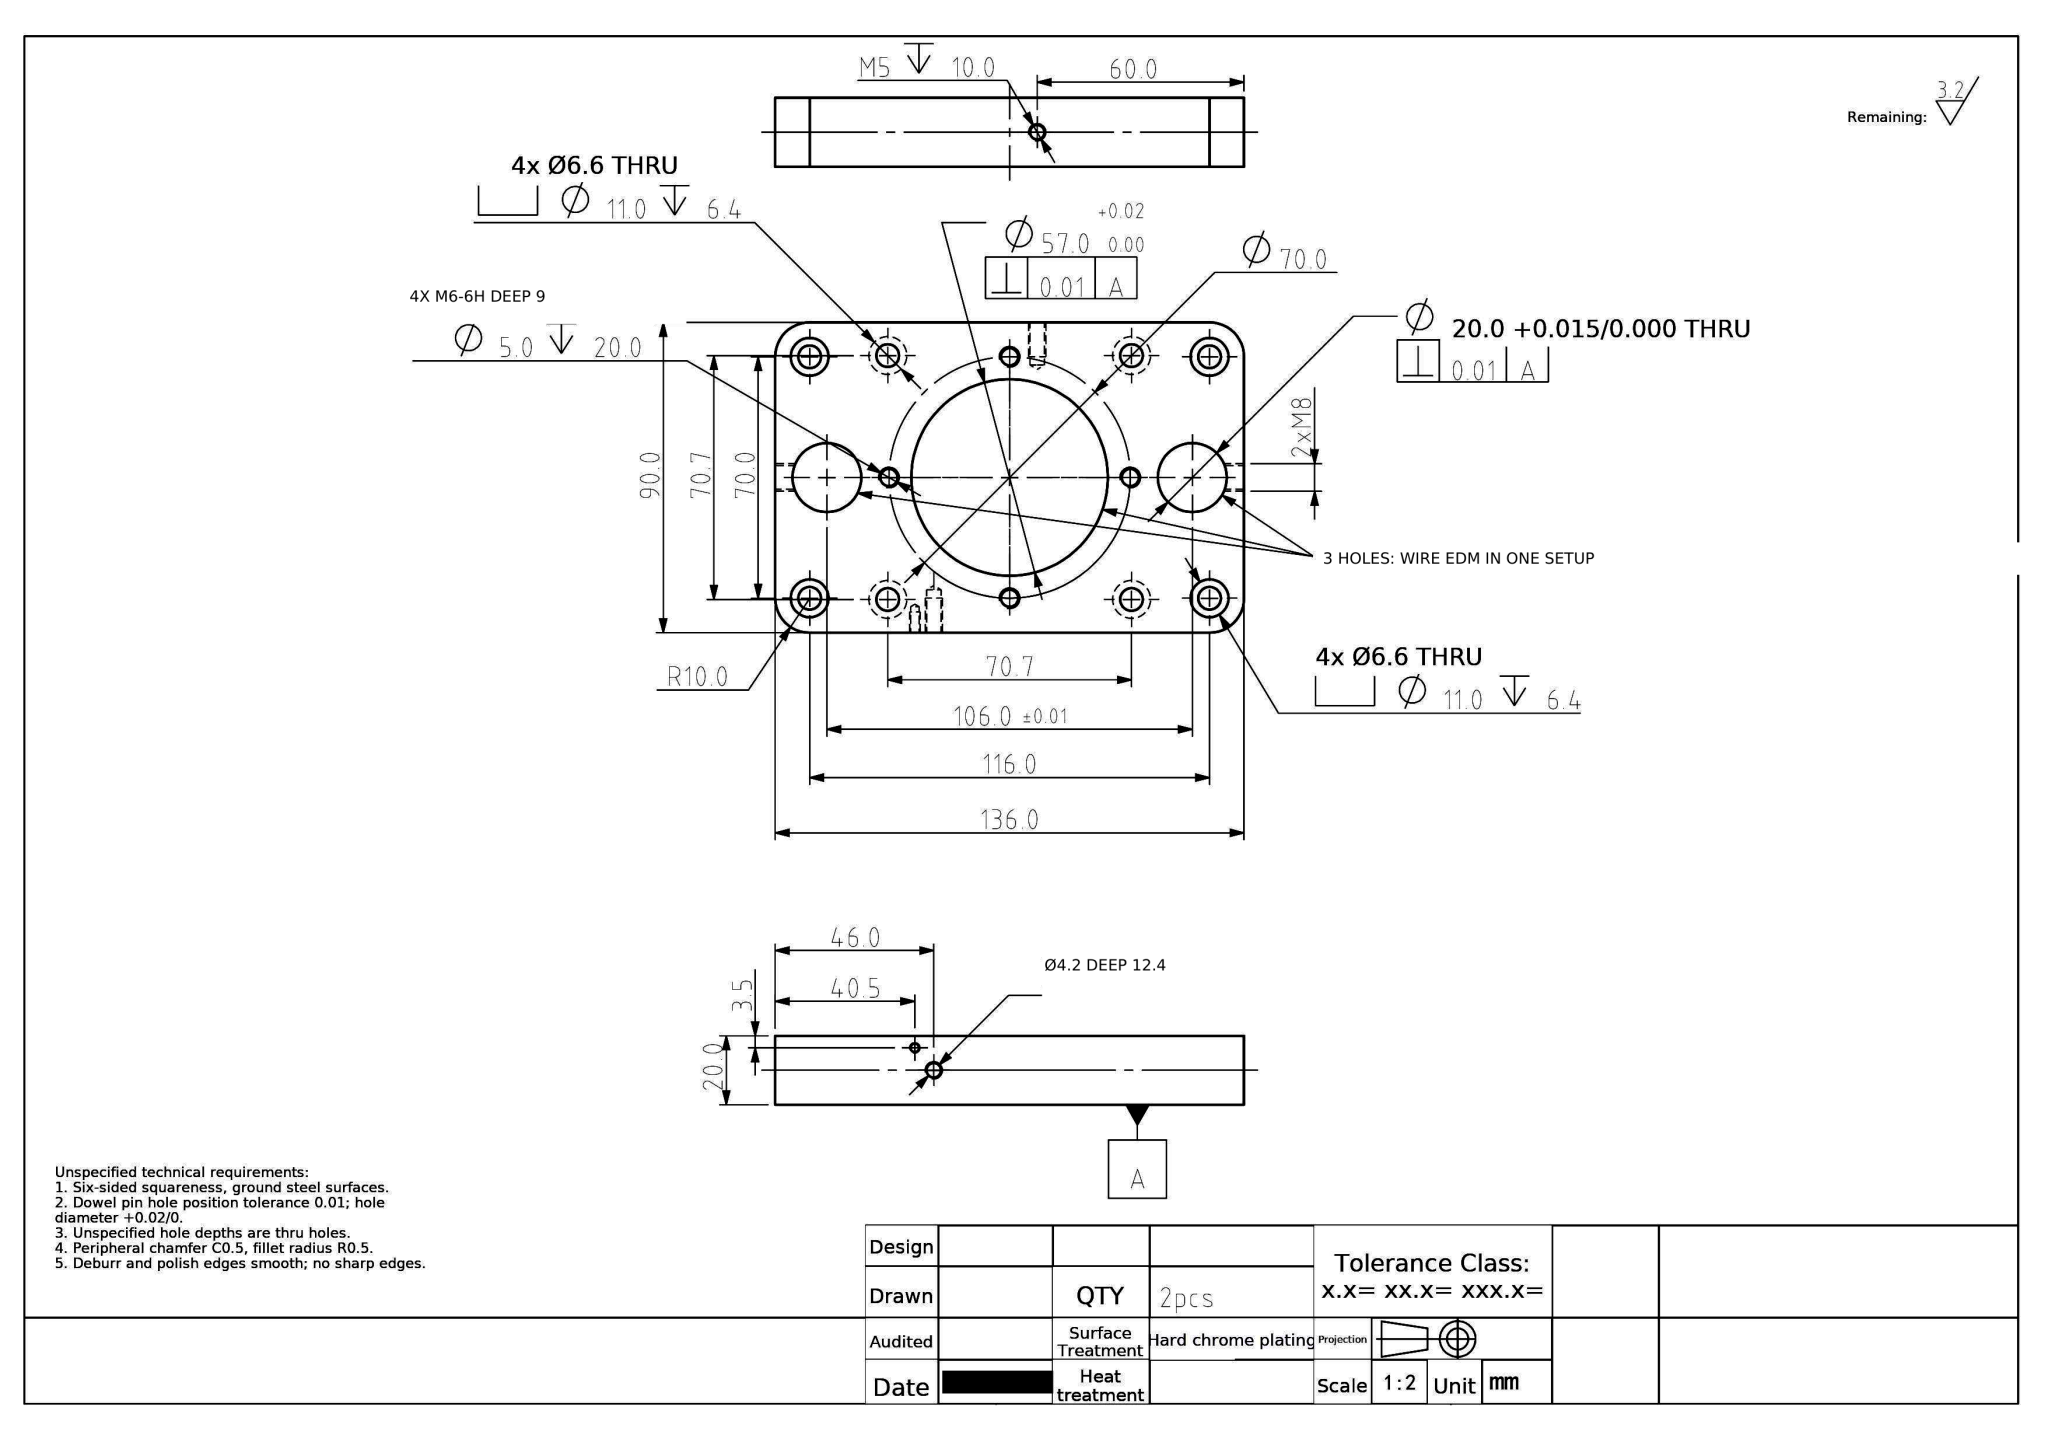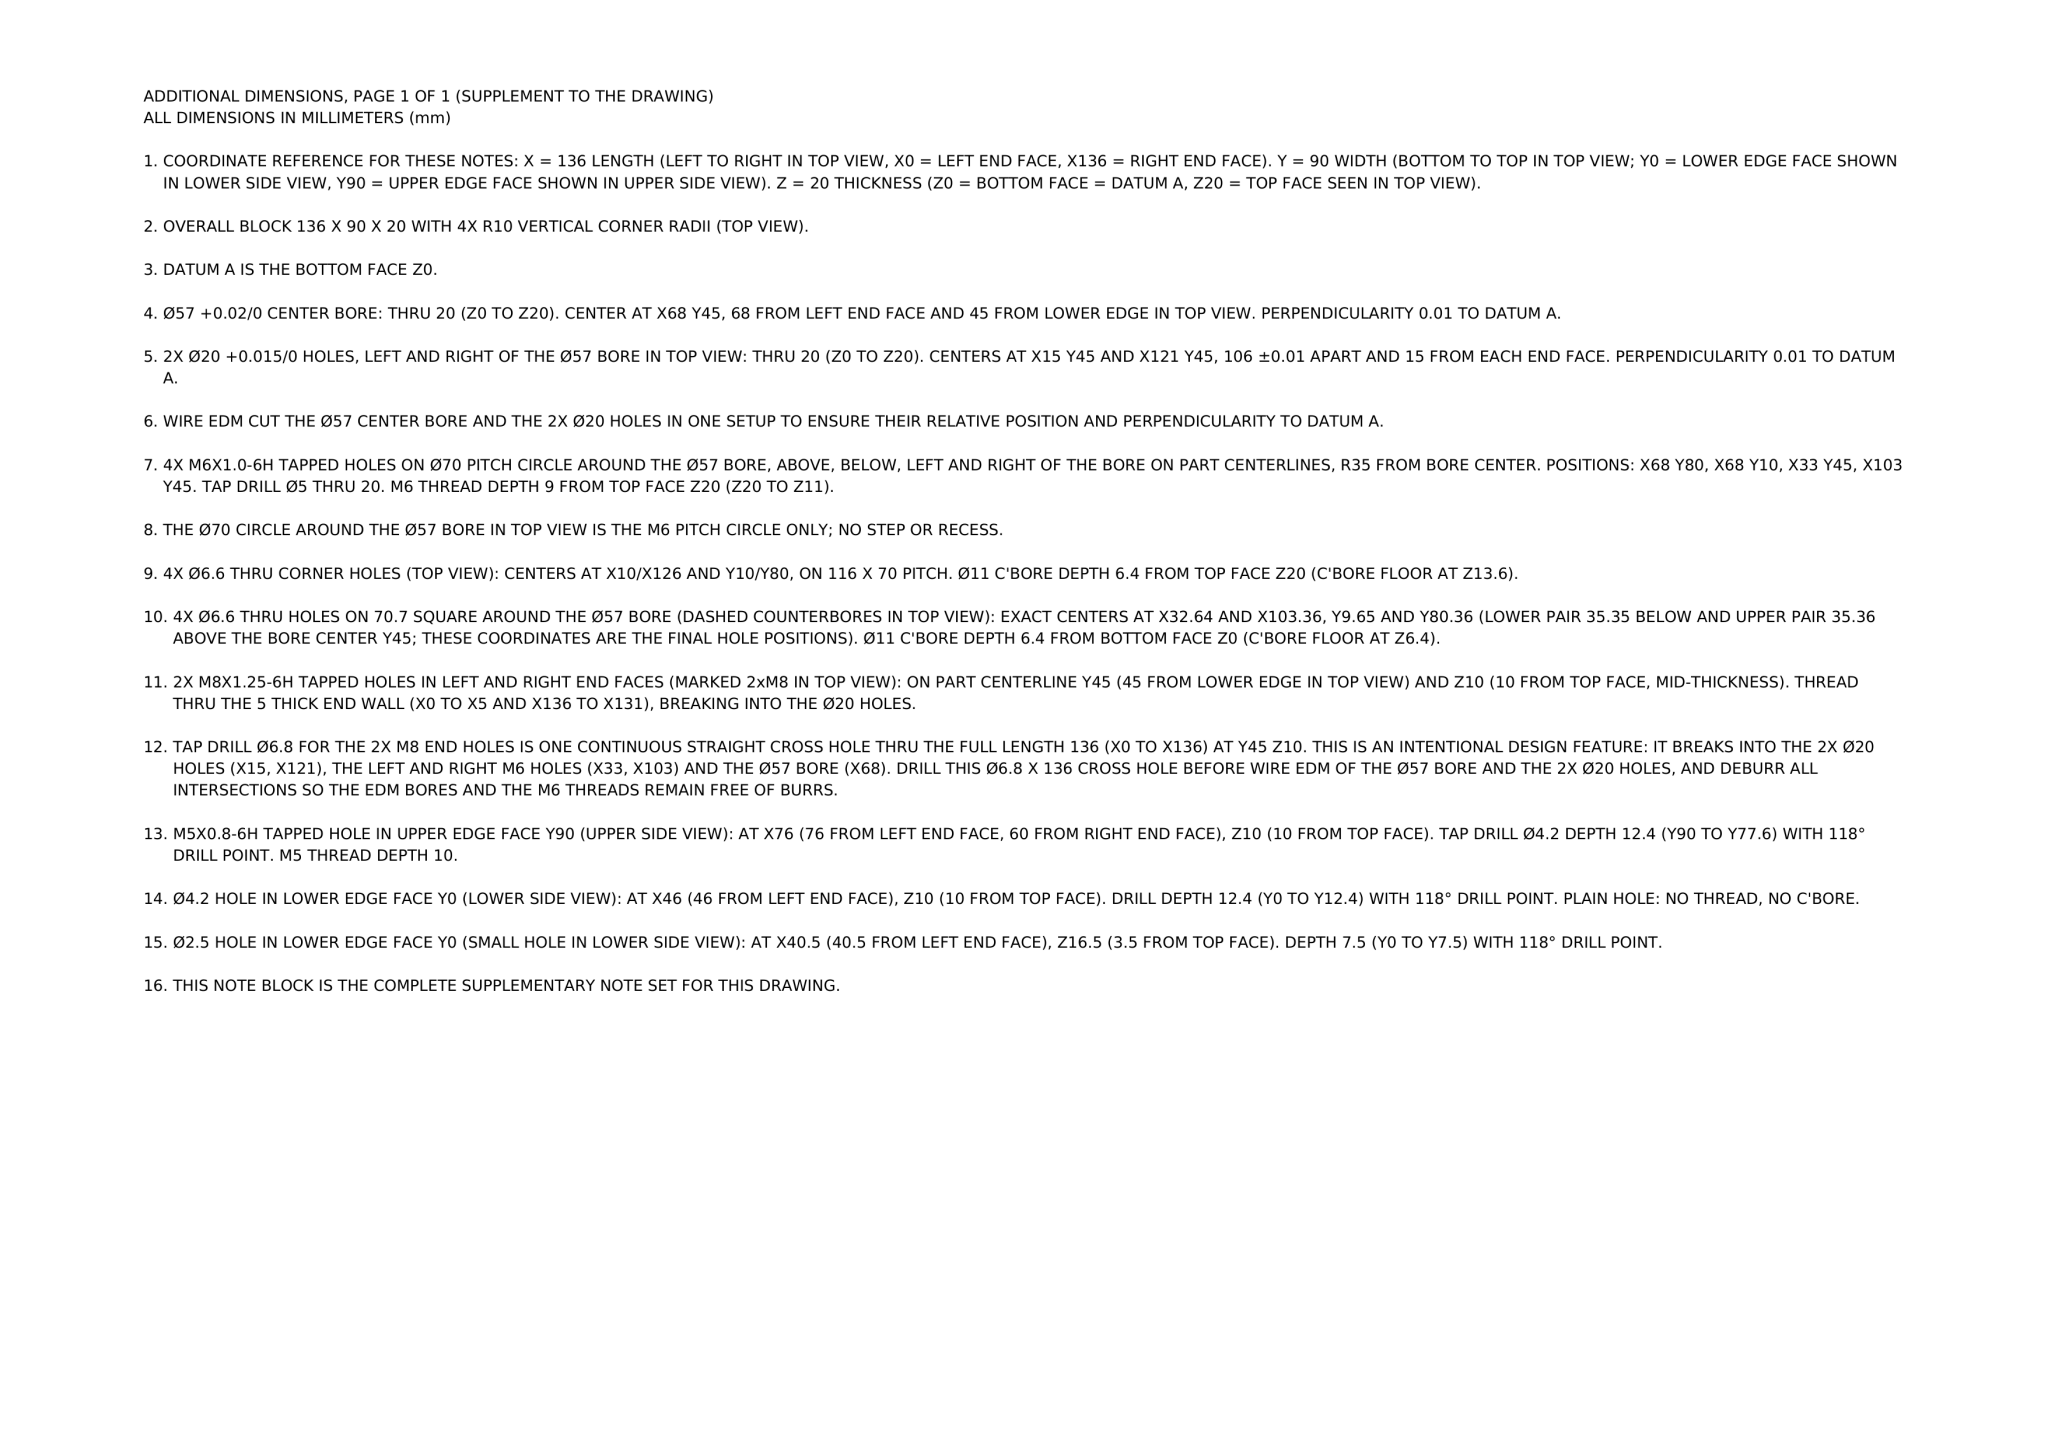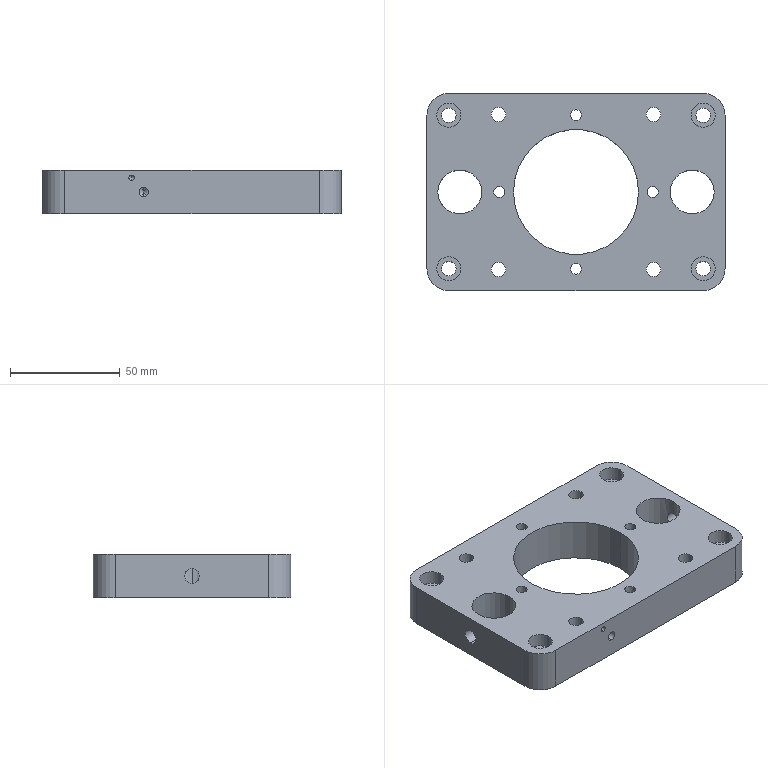Part | NX | mm | 1 solid | 80 faces | box 136 x 90 x 20 mm | volume 168556 mm3 | cylinder 60 | plane 14 | cone 6 | commonest cylinder face diameters 11 x16 6.6 x16 5 x8 20 x8 4.2 x4 6.8 x4 2.5 x2 57 x2